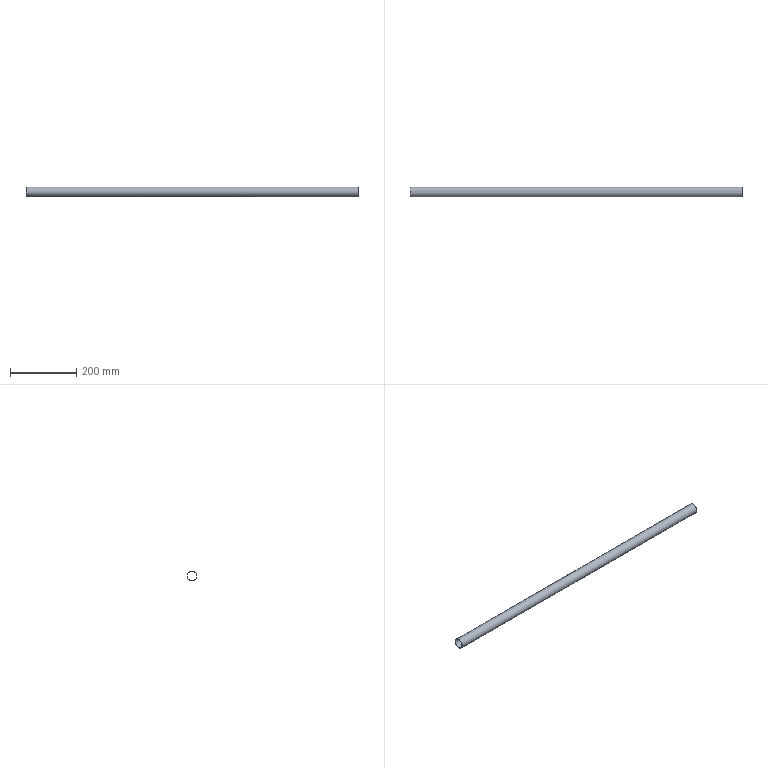Component | SolidWorks | StainlessSteelAxis-1 | 1 solid | 6 faces | box 1000 x 30 x 30 mm | volume 91106 mm3 | cylinder 4 | plane 2 | commonest cylinder face diameters 28 x2 30 x2
build123d program:
from build123d import *

# Parameters (mm, degrees)
SKETCH1_R           = 15
SKETCH1_R_2         = 14
BOSS_EXTRUDE1_DEPTH = 1000


with BuildPart() as part:
    # Sketch1 → Boss-Extrude1 (new body)
    with BuildSketch(Plane.XY):
        Circle(SKETCH1_R)
        Circle(SKETCH1_R_2, mode=Mode.SUBTRACT)
    extrude(amount=BOSS_EXTRUDE1_DEPTH)


solid = part.part

# Placed as in the assembly
solid = solid.moved(Location((-65.532, -310.334, 1321.399), (0, 90, 0)))
STEP:
#1=COLOUR_RGB('',0.7922,0.8196,0.9333);
#2=FILL_AREA_STYLE_COLOUR('',#1);
#3=FILL_AREA_STYLE('',(#2));
#4=SURFACE_STYLE_FILL_AREA(#3);
#5=SURFACE_SIDE_STYLE('',(#4));
#6=SURFACE_STYLE_USAGE(.BOTH.,#5);
#7=PRESENTATION_STYLE_ASSIGNMENT((#6));
#8=CARTESIAN_POINT('',(-2.58,-12.532,51.571));
#9=VERTEX_POINT('',#8);
#10=CARTESIAN_POINT('',(-2.58,-11.904,52.476));
#11=VERTEX_POINT('',#10);
#12=CARTESIAN_POINT('',(-2.58,-12.218,52.024));
#13=DIRECTION('',(-1.,0.,-0.));
#14=DIRECTION('',(-0.,0.5699,0.8217));
#15=AXIS2_PLACEMENT_3D('',#12,#13,#14);
#16=CIRCLE('',#15,0.5512);
#17=EDGE_CURVE('',#9,#11,#16,.T.);
#18=ORIENTED_EDGE('',*,*,#17,.T.);
#19=CARTESIAN_POINT('',(36.79,-11.904,52.476));
#20=VERTEX_POINT('',#19);
#21=CARTESIAN_POINT('',(-2.58,-11.904,52.476));
#22=DIRECTION('',(1.,-0.,0.));
#23=VECTOR('',#22,39.37);
#24=LINE('',#21,#23);
#25=EDGE_CURVE('',#11,#20,#24,.T.);
#26=ORIENTED_EDGE('',*,*,#25,.T.);
#27=CARTESIAN_POINT('',(36.79,-12.532,51.571));
#28=VERTEX_POINT('',#27);
#29=CARTESIAN_POINT('',(36.79,-12.218,52.024));
#30=DIRECTION('',(-1.,0.,-0.));
#31=DIRECTION('',(0.,0.5699,0.8217));
#32=AXIS2_PLACEMENT_3D('',#29,#30,#31);
#33=CIRCLE('',#32,0.5512);
#34=EDGE_CURVE('',#28,#20,#33,.T.);
#35=ORIENTED_EDGE('',*,*,#34,.F.);
#36=CARTESIAN_POINT('',(-2.58,-12.532,51.571));
#37=DIRECTION('',(1.,-0.,0.));
#38=VECTOR('',#37,39.37);
#39=LINE('',#36,#38);
#40=EDGE_CURVE('',#9,#28,#39,.T.);
#41=ORIENTED_EDGE('',*,*,#40,.F.);
#42=EDGE_LOOP('',(#18,#26,#35,#41));
#43=FACE_OUTER_BOUND('',#42,.T.);
#44=CARTESIAN_POINT('',(-2.58,-12.218,52.024));
#45=DIRECTION('',(1.,-0.,0.));
#46=DIRECTION('',(0.,-0.5699,-0.8217));
#47=AXIS2_PLACEMENT_3D('',#44,#45,#46);
#48=CYLINDRICAL_SURFACE('',#47,0.5512);
#49=ADVANCED_FACE('',(#43),#48,.F.);
#50=CARTESIAN_POINT('',(-2.58,-11.881,52.509));
#51=VERTEX_POINT('',#50);
#52=CARTESIAN_POINT('',(-2.58,-12.554,51.538));
#53=VERTEX_POINT('',#52);
#54=CARTESIAN_POINT('',(-2.58,-12.218,52.024));
#55=DIRECTION('',(-1.,0.,-0.));
#56=DIRECTION('',(-0.,0.5699,0.8217));
#57=AXIS2_PLACEMENT_3D('',#54,#55,#56);
#58=CIRCLE('',#57,0.5906);
#59=EDGE_CURVE('',#51,#53,#58,.T.);
#60=ORIENTED_EDGE('',*,*,#59,.F.);
#61=CARTESIAN_POINT('',(36.79,-11.881,52.509));
#62=VERTEX_POINT('',#61);
#63=CARTESIAN_POINT('',(-2.58,-11.881,52.509));
#64=DIRECTION('',(1.,-0.,0.));
#65=VECTOR('',#64,39.37);
#66=LINE('',#63,#65);
#67=EDGE_CURVE('',#51,#62,#66,.T.);
#68=ORIENTED_EDGE('',*,*,#67,.T.);
#69=CARTESIAN_POINT('',(36.79,-12.554,51.538));
#70=VERTEX_POINT('',#69);
#71=CARTESIAN_POINT('',(36.79,-12.218,52.024));
#72=DIRECTION('',(-1.,0.,-0.));
#73=DIRECTION('',(0.,0.5699,0.8217));
#74=AXIS2_PLACEMENT_3D('',#71,#72,#73);
#75=CIRCLE('',#74,0.5906);
#76=EDGE_CURVE('',#62,#70,#75,.T.);
#77=ORIENTED_EDGE('',*,*,#76,.T.);
#78=CARTESIAN_POINT('',(-2.58,-12.554,51.538));
#79=DIRECTION('',(1.,-0.,0.));
#80=VECTOR('',#79,39.37);
#81=LINE('',#78,#80);
#82=EDGE_CURVE('',#53,#70,#81,.T.);
#83=ORIENTED_EDGE('',*,*,#82,.F.);
#84=EDGE_LOOP('',(#60,#68,#77,#83));
#85=FACE_OUTER_BOUND('',#84,.T.);
#86=CARTESIAN_POINT('',(-2.58,-12.218,52.024));
#87=DIRECTION('',(1.,-0.,0.));
#88=DIRECTION('',(0.,-0.5699,-0.8217));
#89=AXIS2_PLACEMENT_3D('',#86,#87,#88);
#90=CYLINDRICAL_SURFACE('',#89,0.5906);
#91=ADVANCED_FACE('',(#85),#90,.T.);
#92=CARTESIAN_POINT('',(-2.58,-12.218,52.024));
#93=DIRECTION('',(-1.,0.,-0.));
#94=DIRECTION('',(-0.,0.5699,0.8217));
#95=AXIS2_PLACEMENT_3D('',#92,#93,#94);
#96=CIRCLE('',#95,0.5906);
#97=EDGE_CURVE('',#53,#51,#96,.T.);
#98=ORIENTED_EDGE('',*,*,#97,.T.);
#99=ORIENTED_EDGE('',*,*,#59,.T.);
#100=EDGE_LOOP('',(#98,#99));
#101=FACE_OUTER_BOUND('',#100,.T.);
#102=ORIENTED_EDGE('',*,*,#17,.F.);
#103=CARTESIAN_POINT('',(-2.58,-12.218,52.024));
#104=DIRECTION('',(-1.,0.,-0.));
#105=DIRECTION('',(-0.,0.5699,0.8217));
#106=AXIS2_PLACEMENT_3D('',#103,#104,#105);
#107=CIRCLE('',#106,0.5512);
#108=EDGE_CURVE('',#11,#9,#107,.T.);
#109=ORIENTED_EDGE('',*,*,#108,.F.);
#110=EDGE_LOOP('',(#102,#109));
#111=FACE_BOUND('',#110,.T.);
#112=CARTESIAN_POINT('',(-2.58,-12.218,52.024));
#113=DIRECTION('',(-1.,0.,-0.));
#114=DIRECTION('',(-0.,0.5699,0.8217));
#115=AXIS2_PLACEMENT_3D('',#112,#113,#114);
#116=PLANE('',#115);
#117=ADVANCED_FACE('',(#101,#111),#116,.T.);
#118=CARTESIAN_POINT('',(36.79,-12.218,52.024));
#119=DIRECTION('',(-1.,0.,-0.));
#120=DIRECTION('',(0.,0.5699,0.8217));
#121=AXIS2_PLACEMENT_3D('',#118,#119,#120);
#122=CIRCLE('',#121,0.5906);
#123=EDGE_CURVE('',#70,#62,#122,.T.);
#124=ORIENTED_EDGE('',*,*,#123,.F.);
#125=ORIENTED_EDGE('',*,*,#76,.F.);
#126=EDGE_LOOP('',(#124,#125));
#127=FACE_OUTER_BOUND('',#126,.T.);
#128=ORIENTED_EDGE('',*,*,#34,.T.);
#129=CARTESIAN_POINT('',(36.79,-12.218,52.024));
#130=DIRECTION('',(-1.,0.,-0.));
#131=DIRECTION('',(0.,0.5699,0.8217));
#132=AXIS2_PLACEMENT_3D('',#129,#130,#131);
#133=CIRCLE('',#132,0.5512);
#134=EDGE_CURVE('',#20,#28,#133,.T.);
#135=ORIENTED_EDGE('',*,*,#134,.T.);
#136=EDGE_LOOP('',(#128,#135));
#137=FACE_BOUND('',#136,.T.);
#138=CARTESIAN_POINT('',(36.79,-12.218,52.024));
#139=DIRECTION('',(-1.,0.,-0.));
#140=DIRECTION('',(-0.,0.5699,0.8217));
#141=AXIS2_PLACEMENT_3D('',#138,#139,#140);
#142=PLANE('',#141);
#143=ADVANCED_FACE('',(#127,#137),#142,.F.);
#144=ORIENTED_EDGE('',*,*,#67,.F.);
#145=ORIENTED_EDGE('',*,*,#97,.F.);
#146=ORIENTED_EDGE('',*,*,#82,.T.);
#147=ORIENTED_EDGE('',*,*,#123,.T.);
#148=EDGE_LOOP('',(#144,#145,#146,#147));
#149=FACE_OUTER_BOUND('',#148,.T.);
#150=CARTESIAN_POINT('',(-2.58,-12.218,52.024));
#151=DIRECTION('',(1.,-0.,0.));
#152=DIRECTION('',(0.,-0.5699,-0.8217));
#153=AXIS2_PLACEMENT_3D('',#150,#151,#152);
#154=CYLINDRICAL_SURFACE('',#153,0.5906);
#155=ADVANCED_FACE('',(#149),#154,.T.);
#156=ORIENTED_EDGE('',*,*,#25,.F.);
#157=ORIENTED_EDGE('',*,*,#108,.T.);
#158=ORIENTED_EDGE('',*,*,#40,.T.);
#159=ORIENTED_EDGE('',*,*,#134,.F.);
#160=EDGE_LOOP('',(#156,#157,#158,#159));
#161=FACE_OUTER_BOUND('',#160,.T.);
#162=CARTESIAN_POINT('',(-2.58,-12.218,52.024));
#163=DIRECTION('',(1.,-0.,0.));
#164=DIRECTION('',(0.,-0.5699,-0.8217));
#165=AXIS2_PLACEMENT_3D('',#162,#163,#164);
#166=CYLINDRICAL_SURFACE('',#165,0.5512);
#167=ADVANCED_FACE('',(#161),#166,.F.);
#168=CLOSED_SHELL('',(#49,#91,#117,#143,#155,#167));
#169=MANIFOLD_SOLID_BREP('',#168);
#170=STYLED_ITEM('',(#7),#169);
#171=(LENGTH_UNIT()NAMED_UNIT(*)SI_UNIT($,.METRE.));
#172=LENGTH_MEASURE_WITH_UNIT(LENGTH_MEASURE(0.0254),#171);
#173=DIMENSIONAL_EXPONENTS(1.,0.,0.,0.,0.,0.,0.);
#174=(CONVERSION_BASED_UNIT('',#172)LENGTH_UNIT()NAMED_UNIT(#173));
#175=UNCERTAINTY_MEASURE_WITH_UNIT(LENGTH_MEASURE(0.00001),#174,'','');
#176=(NAMED_UNIT(*)PLANE_ANGLE_UNIT()SI_UNIT($,.RADIAN.));
#177=(NAMED_UNIT(*)SI_UNIT($,.STERADIAN.)SOLID_ANGLE_UNIT());
#178=(GEOMETRIC_REPRESENTATION_CONTEXT(3)GLOBAL_UNCERTAINTY_ASSIGNED_CONTEXT((#175))GLOBAL_UNIT_ASSIGNED_CONTEXT((#174,#176,#177))REPRESENTATION_CONTEXT('',''));
#179=MECHANICAL_DESIGN_GEOMETRIC_PRESENTATION_REPRESENTATION('',(#170),#178);
#180=PRESENTATION_LAYER_ASSIGNMENT('','',(#170));
#181=CARTESIAN_POINT('',(0.,0.,0.));
#182=DIRECTION('',(0.,0.,1.));
#183=DIRECTION('',(1.,0.,0.));
#184=AXIS2_PLACEMENT_3D('',#181,#182,#183);
#185=(LENGTH_UNIT()NAMED_UNIT(*)SI_UNIT($,.METRE.));
#186=LENGTH_MEASURE_WITH_UNIT(LENGTH_MEASURE(0.0254),#185);
#187=DIMENSIONAL_EXPONENTS(1.,0.,0.,0.,0.,0.,0.);
#188=(CONVERSION_BASED_UNIT('',#186)LENGTH_UNIT()NAMED_UNIT(#187));
#189=UNCERTAINTY_MEASURE_WITH_UNIT(LENGTH_MEASURE(0.00001),#188,'','');
#190=(NAMED_UNIT(*)PLANE_ANGLE_UNIT()SI_UNIT($,.RADIAN.));
#191=(NAMED_UNIT(*)SI_UNIT($,.STERADIAN.)SOLID_ANGLE_UNIT());
#192=(GEOMETRIC_REPRESENTATION_CONTEXT(3)GLOBAL_UNCERTAINTY_ASSIGNED_CONTEXT((#189))GLOBAL_UNIT_ASSIGNED_CONTEXT((#188,#190,#191))REPRESENTATION_CONTEXT('',''));
#193=ADVANCED_BREP_SHAPE_REPRESENTATION('',(#169,#184),#192);